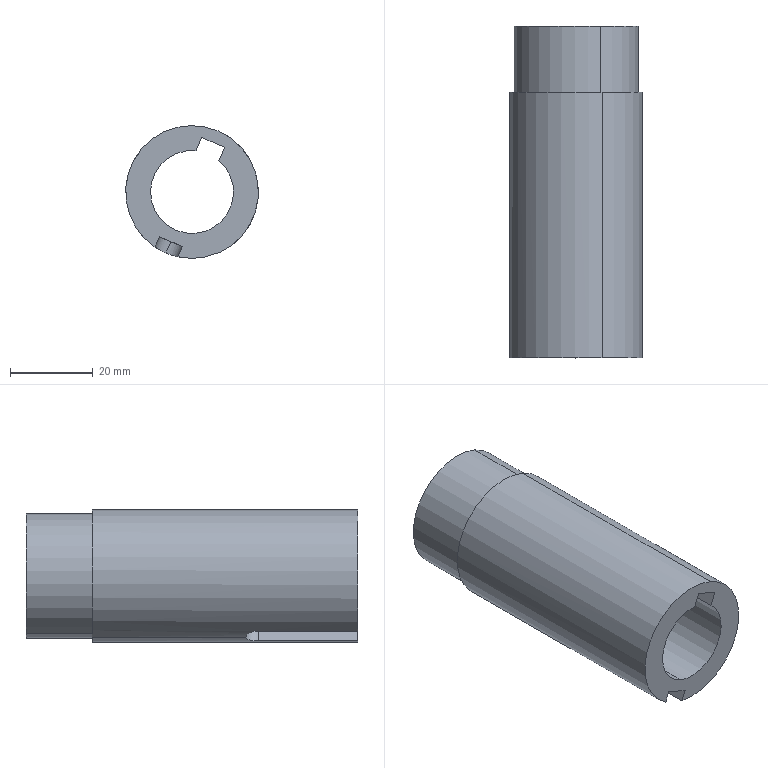Component | SolidWorks | -MovingSleeve-1 | 1 solid | 17 faces | box 32 x 80 x 32 mm | volume 35676 mm3 | plane 9 | cylinder 8 | commonest cylinder face diameters 6 x2 32 x2 30 x2 20 x2
build123d program:
from build123d import *

# Parameters (mm, degrees)
CUT_EXTRUDE1_DEPTH = 3
SKETCH3_W          = 6.215
SKETCH3_H          = 6
CUT_EXTRUDE2_DEPTH = 84.138


with BuildPart() as part:
    # Sketch1 → Revolve1 (revolve)
    with BuildSketch(Plane.XY):
        Polygon((15, 80), (15, 64), (16, 64), (16, 48), (16, 38), (16, 0), (10, 0), (10, 80), align=None)
    revolve(axis=Axis((0, -3319.583, 0), (0, 1, 0)))

    # Sketch2 → Cut-Extrude1 (cut)
    with BuildSketch(Plane(origin=(16, 0, 0), x_dir=(0, 0, -1), z_dir=(1, 0, 0))):
        with BuildLine():
            Line((-3, 0), (-3, 24))
            ThreePointArc((-3, 24), (0, 27), (3, 24))
            Line((3, 24), (3, 0))
            ThreePointArc((3, 0), (0, -3), (-3, 0))
        make_face()
    extrude(amount=-CUT_EXTRUDE1_DEPTH, mode=Mode.SUBTRACT)

    # Sketch3 → Cut-Extrude2 (cut, through all)
    with BuildSketch(Plane.XZ):
        with Locations((-9.893, 0)):
            Rectangle(SKETCH3_W, SKETCH3_H)
    extrude(amount=-CUT_EXTRUDE2_DEPTH, mode=Mode.SUBTRACT)


solid = part.part

# Placed as in the assembly
solid = solid.moved(Location((205, 1261.878, -173), (180, 66.949, -180)))
STEP:
#1=COLOUR_RGB('',0.7922,0.8196,0.9333);
#2=FILL_AREA_STYLE_COLOUR('',#1);
#3=FILL_AREA_STYLE('',(#2));
#4=SURFACE_STYLE_FILL_AREA(#3);
#5=SURFACE_SIDE_STYLE('',(#4));
#6=SURFACE_STYLE_USAGE(.BOTH.,#5);
#7=PRESENTATION_STYLE_ASSIGNMENT((#6));
#8=CARTESIAN_POINT('',(7.87,50.743,-7.282));
#9=VERTEX_POINT('',#8);
#10=CARTESIAN_POINT('',(7.979,50.625,-7.328));
#11=VERTEX_POINT('',#10);
#12=CARTESIAN_POINT('',(7.87,50.625,-7.282));
#13=DIRECTION('',(-0.3916,0.,-0.9202));
#14=DIRECTION('',(0.,1.,0.));
#15=AXIS2_PLACEMENT_3D('',#12,#13,#14);
#16=CIRCLE('',#15,0.1181);
#17=EDGE_CURVE('',#9,#11,#16,.T.);
#18=ORIENTED_EDGE('',*,*,#17,.F.);
#19=CARTESIAN_POINT('',(7.824,50.743,-7.391));
#20=VERTEX_POINT('',#19);
#21=CARTESIAN_POINT('',(7.87,50.743,-7.282));
#22=DIRECTION('',(-0.3916,0.,-0.9202));
#23=VECTOR('',#22,39.37);
#24=LINE('',#21,#23);
#25=EDGE_CURVE('',#9,#20,#24,.T.);
#26=ORIENTED_EDGE('',*,*,#25,.T.);
#27=CARTESIAN_POINT('',(7.937,50.625,-7.427));
#28=VERTEX_POINT('',#27);
#29=CARTESIAN_POINT('',(7.824,50.743,-7.391));
#30=CARTESIAN_POINT('',(7.831,50.743,-7.394));
#31=CARTESIAN_POINT('',(7.839,50.742,-7.397));
#32=CARTESIAN_POINT('',(7.853,50.739,-7.402));
#33=CARTESIAN_POINT('',(7.86,50.737,-7.405));
#34=CARTESIAN_POINT('',(7.873,50.731,-7.409));
#35=CARTESIAN_POINT('',(7.88,50.728,-7.411));
#36=CARTESIAN_POINT('',(7.892,50.719,-7.415));
#37=CARTESIAN_POINT('',(7.898,50.714,-7.417));
#38=CARTESIAN_POINT('',(7.909,50.703,-7.42));
#39=CARTESIAN_POINT('',(7.913,50.697,-7.421));
#40=CARTESIAN_POINT('',(7.922,50.684,-7.423));
#41=CARTESIAN_POINT('',(7.925,50.678,-7.424));
#42=CARTESIAN_POINT('',(7.931,50.663,-7.425));
#43=CARTESIAN_POINT('',(7.933,50.656,-7.426));
#44=CARTESIAN_POINT('',(7.936,50.641,-7.426));
#45=CARTESIAN_POINT('',(7.937,50.633,-7.427));
#46=CARTESIAN_POINT('',(7.937,50.625,-7.427));
#47=B_SPLINE_CURVE_WITH_KNOTS('',3,(#29,#30,#31,#32,#33,#34,#35,#36,#37,#38,#39,#40,#41,#42,#43,#44,#45,#46),.UNSPECIFIED.,.F.,.F.,(4,2,2,2,2,2,2,2,4),(0.004701,0.005288,0.005875,0.006462,0.007049,0.007637,0.008224,0.008811,0.009398),.UNSPECIFIED.);
#48=EDGE_CURVE('',#20,#28,#47,.T.);
#49=ORIENTED_EDGE('',*,*,#48,.T.);
#50=CARTESIAN_POINT('',(7.979,50.625,-7.328));
#51=DIRECTION('',(-0.3916,0.,-0.9202));
#52=VECTOR('',#51,39.37);
#53=LINE('',#50,#52);
#54=EDGE_CURVE('',#11,#28,#53,.T.);
#55=ORIENTED_EDGE('',*,*,#54,.F.);
#56=EDGE_LOOP('',(#18,#26,#49,#55));
#57=FACE_OUTER_BOUND('',#56,.T.);
#58=CARTESIAN_POINT('',(7.87,50.625,-7.282));
#59=DIRECTION('',(-0.3916,0.,-0.9202));
#60=DIRECTION('',(0.,1.,0.));
#61=AXIS2_PLACEMENT_3D('',#58,#59,#60);
#62=CYLINDRICAL_SURFACE('',#61,0.1181);
#63=ADVANCED_FACE('',(#57),#62,.F.);
#64=CARTESIAN_POINT('',(7.824,52.2,-7.391));
#65=VERTEX_POINT('',#64);
#66=CARTESIAN_POINT('',(8.318,52.2,-6.231));
#67=VERTEX_POINT('',#66);
#68=CARTESIAN_POINT('',(8.071,52.2,-6.811));
#69=DIRECTION('',(-0.,-1.,-0.));
#70=DIRECTION('',(-0.3916,0.,-0.9202));
#71=AXIS2_PLACEMENT_3D('',#68,#69,#70);
#72=CIRCLE('',#71,0.6299);
#73=EDGE_CURVE('',#65,#67,#72,.T.);
#74=ORIENTED_EDGE('',*,*,#73,.T.);
#75=CARTESIAN_POINT('',(8.318,49.68,-6.231));
#76=VERTEX_POINT('',#75);
#77=CARTESIAN_POINT('',(8.318,-81.012,-6.231));
#78=DIRECTION('',(-0.,-1.,-0.));
#79=VECTOR('',#78,39.37);
#80=LINE('',#77,#79);
#81=EDGE_CURVE('',#67,#76,#80,.T.);
#82=ORIENTED_EDGE('',*,*,#81,.T.);
#83=CARTESIAN_POINT('',(7.937,49.68,-7.427));
#84=VERTEX_POINT('',#83);
#85=CARTESIAN_POINT('',(8.071,49.68,-6.811));
#86=DIRECTION('',(-0.,-1.,-0.));
#87=DIRECTION('',(-0.3916,0.,-0.9202));
#88=AXIS2_PLACEMENT_3D('',#85,#86,#87);
#89=CIRCLE('',#88,0.6299);
#90=EDGE_CURVE('',#84,#76,#89,.T.);
#91=ORIENTED_EDGE('',*,*,#90,.F.);
#92=CARTESIAN_POINT('',(7.937,-81.012,-7.427));
#93=DIRECTION('',(-0.,-1.,-0.));
#94=VECTOR('',#93,39.37);
#95=LINE('',#92,#94);
#96=EDGE_CURVE('',#28,#84,#95,.T.);
#97=ORIENTED_EDGE('',*,*,#96,.F.);
#98=ORIENTED_EDGE('',*,*,#48,.F.);
#99=CARTESIAN_POINT('',(7.824,-81.012,-7.391));
#100=DIRECTION('',(-0.,-1.,-0.));
#101=VECTOR('',#100,39.37);
#102=LINE('',#99,#101);
#103=EDGE_CURVE('',#65,#20,#102,.T.);
#104=ORIENTED_EDGE('',*,*,#103,.F.);
#105=EDGE_LOOP('',(#74,#82,#91,#97,#98,#104));
#106=FACE_OUTER_BOUND('',#105,.T.);
#107=CARTESIAN_POINT('',(8.071,-81.012,-6.811));
#108=DIRECTION('',(-0.,-1.,-0.));
#109=DIRECTION('',(-0.3916,0.,-0.9202));
#110=AXIS2_PLACEMENT_3D('',#107,#108,#109);
#111=CYLINDRICAL_SURFACE('',#110,0.6299);
#112=ADVANCED_FACE('',(#106),#111,.T.);
#113=CARTESIAN_POINT('',(7.84,52.83,-7.354));
#114=VERTEX_POINT('',#113);
#115=CARTESIAN_POINT('',(8.302,52.83,-6.268));
#116=VERTEX_POINT('',#115);
#117=CARTESIAN_POINT('',(8.071,52.83,-6.811));
#118=DIRECTION('',(-0.,-1.,-0.));
#119=DIRECTION('',(-0.3916,0.,-0.9202));
#120=AXIS2_PLACEMENT_3D('',#117,#118,#119);
#121=CIRCLE('',#120,0.5906);
#122=EDGE_CURVE('',#114,#116,#121,.T.);
#123=ORIENTED_EDGE('',*,*,#122,.T.);
#124=CARTESIAN_POINT('',(8.302,52.2,-6.268));
#125=VERTEX_POINT('',#124);
#126=CARTESIAN_POINT('',(8.302,-81.012,-6.268));
#127=DIRECTION('',(-0.,-1.,-0.));
#128=VECTOR('',#127,39.37);
#129=LINE('',#126,#128);
#130=EDGE_CURVE('',#116,#125,#129,.T.);
#131=ORIENTED_EDGE('',*,*,#130,.T.);
#132=CARTESIAN_POINT('',(7.84,52.2,-7.354));
#133=VERTEX_POINT('',#132);
#134=CARTESIAN_POINT('',(8.071,52.2,-6.811));
#135=DIRECTION('',(-0.,-1.,-0.));
#136=DIRECTION('',(-0.3916,0.,-0.9202));
#137=AXIS2_PLACEMENT_3D('',#134,#135,#136);
#138=CIRCLE('',#137,0.5906);
#139=EDGE_CURVE('',#133,#125,#138,.T.);
#140=ORIENTED_EDGE('',*,*,#139,.F.);
#141=CARTESIAN_POINT('',(7.84,-81.012,-7.354));
#142=DIRECTION('',(-0.,-1.,-0.));
#143=VECTOR('',#142,39.37);
#144=LINE('',#141,#143);
#145=EDGE_CURVE('',#114,#133,#144,.T.);
#146=ORIENTED_EDGE('',*,*,#145,.F.);
#147=EDGE_LOOP('',(#123,#131,#140,#146));
#148=FACE_OUTER_BOUND('',#147,.T.);
#149=CARTESIAN_POINT('',(8.071,-81.012,-6.811));
#150=DIRECTION('',(-0.,-1.,-0.));
#151=DIRECTION('',(-0.3916,0.,-0.9202));
#152=AXIS2_PLACEMENT_3D('',#149,#150,#151);
#153=CYLINDRICAL_SURFACE('',#152,0.5906);
#154=ADVANCED_FACE('',(#148),#153,.T.);
#155=CARTESIAN_POINT('',(7.917,52.83,-7.173));
#156=VERTEX_POINT('',#155);
#157=CARTESIAN_POINT('',(8.327,52.83,-6.512));
#158=VERTEX_POINT('',#157);
#159=CARTESIAN_POINT('',(8.071,52.83,-6.811));
#160=DIRECTION('',(-0.,-1.,-0.));
#161=DIRECTION('',(-0.3916,0.,-0.9202));
#162=AXIS2_PLACEMENT_3D('',#159,#160,#161);
#163=CIRCLE('',#162,0.3937);
#164=EDGE_CURVE('',#156,#158,#163,.T.);
#165=ORIENTED_EDGE('',*,*,#164,.F.);
#166=CARTESIAN_POINT('',(7.917,49.68,-7.173));
#167=VERTEX_POINT('',#166);
#168=CARTESIAN_POINT('',(7.917,-81.012,-7.173));
#169=DIRECTION('',(-0.,-1.,-0.));
#170=VECTOR('',#169,39.37);
#171=LINE('',#168,#170);
#172=EDGE_CURVE('',#156,#167,#171,.T.);
#173=ORIENTED_EDGE('',*,*,#172,.T.);
#174=CARTESIAN_POINT('',(8.327,49.68,-6.512));
#175=VERTEX_POINT('',#174);
#176=CARTESIAN_POINT('',(8.071,49.68,-6.811));
#177=DIRECTION('',(-0.,-1.,-0.));
#178=DIRECTION('',(-0.3916,0.,-0.9202));
#179=AXIS2_PLACEMENT_3D('',#176,#177,#178);
#180=CIRCLE('',#179,0.3937);
#181=EDGE_CURVE('',#167,#175,#180,.T.);
#182=ORIENTED_EDGE('',*,*,#181,.T.);
#183=CARTESIAN_POINT('',(8.327,-81.012,-6.512));
#184=DIRECTION('',(-0.,-1.,-0.));
#185=VECTOR('',#184,39.37);
#186=LINE('',#183,#185);
#187=EDGE_CURVE('',#158,#175,#186,.T.);
#188=ORIENTED_EDGE('',*,*,#187,.F.);
#189=EDGE_LOOP('',(#165,#173,#182,#188));
#190=FACE_OUTER_BOUND('',#189,.T.);
#191=CARTESIAN_POINT('',(8.071,-81.012,-6.811));
#192=DIRECTION('',(-0.,-1.,-0.));
#193=DIRECTION('',(-0.3916,0.,-0.9202));
#194=AXIS2_PLACEMENT_3D('',#191,#192,#193);
#195=CYLINDRICAL_SURFACE('',#194,0.3937);
#196=ADVANCED_FACE('',(#190),#195,.F.);
#197=ORIENTED_EDGE('',*,*,#172,.F.);
#198=CARTESIAN_POINT('',(8.109,52.83,-6.419));
#199=VERTEX_POINT('',#198);
#200=CARTESIAN_POINT('',(8.071,52.83,-6.811));
#201=DIRECTION('',(-0.,-1.,-0.));
#202=DIRECTION('',(-0.3916,0.,-0.9202));
#203=AXIS2_PLACEMENT_3D('',#200,#201,#202);
#204=CIRCLE('',#203,0.3937);
#205=EDGE_CURVE('',#199,#156,#204,.T.);
#206=ORIENTED_EDGE('',*,*,#205,.F.);
#207=CARTESIAN_POINT('',(8.109,49.68,-6.419));
#208=VERTEX_POINT('',#207);
#209=CARTESIAN_POINT('',(8.109,-81.012,-6.419));
#210=DIRECTION('',(0.,1.,0.));
#211=VECTOR('',#210,39.37);
#212=LINE('',#209,#211);
#213=EDGE_CURVE('',#208,#199,#212,.T.);
#214=ORIENTED_EDGE('',*,*,#213,.F.);
#215=CARTESIAN_POINT('',(8.071,49.68,-6.811));
#216=DIRECTION('',(-0.,-1.,-0.));
#217=DIRECTION('',(-0.3916,0.,-0.9202));
#218=AXIS2_PLACEMENT_3D('',#215,#216,#217);
#219=CIRCLE('',#218,0.3937);
#220=EDGE_CURVE('',#208,#167,#219,.T.);
#221=ORIENTED_EDGE('',*,*,#220,.T.);
#222=EDGE_LOOP('',(#197,#206,#214,#221));
#223=FACE_OUTER_BOUND('',#222,.T.);
#224=CARTESIAN_POINT('',(8.071,-81.012,-6.811));
#225=DIRECTION('',(-0.,-1.,-0.));
#226=DIRECTION('',(-0.3916,0.,-0.9202));
#227=AXIS2_PLACEMENT_3D('',#224,#225,#226);
#228=CYLINDRICAL_SURFACE('',#227,0.3937);
#229=ADVANCED_FACE('',(#223),#228,.F.);
#230=CARTESIAN_POINT('',(8.38,52.83,-6.386));
#231=VERTEX_POINT('',#230);
#232=CARTESIAN_POINT('',(8.38,52.83,-6.386));
#233=DIRECTION('',(0.3916,-0.,0.9202));
#234=VECTOR('',#233,39.37);
#235=LINE('',#232,#234);
#236=EDGE_CURVE('',#158,#231,#235,.T.);
#237=ORIENTED_EDGE('',*,*,#236,.T.);
#238=CARTESIAN_POINT('',(8.163,52.83,-6.294));
#239=VERTEX_POINT('',#238);
#240=CARTESIAN_POINT('',(8.38,52.83,-6.386));
#241=DIRECTION('',(-0.9202,0.,0.3916));
#242=VECTOR('',#241,39.37);
#243=LINE('',#240,#242);
#244=EDGE_CURVE('',#231,#239,#243,.T.);
#245=ORIENTED_EDGE('',*,*,#244,.T.);
#246=CARTESIAN_POINT('',(8.163,52.83,-6.294));
#247=DIRECTION('',(-0.3916,0.,-0.9202));
#248=VECTOR('',#247,39.37);
#249=LINE('',#246,#248);
#250=EDGE_CURVE('',#239,#199,#249,.T.);
#251=ORIENTED_EDGE('',*,*,#250,.T.);
#252=ORIENTED_EDGE('',*,*,#205,.T.);
#253=ORIENTED_EDGE('',*,*,#164,.T.);
#254=EDGE_LOOP('',(#237,#245,#251,#252,#253));
#255=FACE_BOUND('',#254,.T.);
#256=ORIENTED_EDGE('',*,*,#122,.F.);
#257=CARTESIAN_POINT('',(8.071,52.83,-6.811));
#258=DIRECTION('',(-0.,-1.,-0.));
#259=DIRECTION('',(-0.3916,0.,-0.9202));
#260=AXIS2_PLACEMENT_3D('',#257,#258,#259);
#261=CIRCLE('',#260,0.5906);
#262=EDGE_CURVE('',#116,#114,#261,.T.);
#263=ORIENTED_EDGE('',*,*,#262,.F.);
#264=EDGE_LOOP('',(#256,#263));
#265=FACE_OUTER_BOUND('',#264,.T.);
#266=CARTESIAN_POINT('',(7.917,52.83,-7.173));
#267=DIRECTION('',(0.,1.,0.));
#268=DIRECTION('',(0.3916,-0.,0.9202));
#269=AXIS2_PLACEMENT_3D('',#266,#267,#268);
#270=PLANE('',#269);
#271=ADVANCED_FACE('',(#255,#265),#270,.T.);
#272=ORIENTED_EDGE('',*,*,#130,.F.);
#273=ORIENTED_EDGE('',*,*,#262,.T.);
#274=ORIENTED_EDGE('',*,*,#145,.T.);
#275=CARTESIAN_POINT('',(8.071,52.2,-6.811));
#276=DIRECTION('',(-0.,-1.,-0.));
#277=DIRECTION('',(-0.3916,0.,-0.9202));
#278=AXIS2_PLACEMENT_3D('',#275,#276,#277);
#279=CIRCLE('',#278,0.5906);
#280=EDGE_CURVE('',#125,#133,#279,.T.);
#281=ORIENTED_EDGE('',*,*,#280,.F.);
#282=EDGE_LOOP('',(#272,#273,#274,#281));
#283=FACE_OUTER_BOUND('',#282,.T.);
#284=CARTESIAN_POINT('',(8.071,-81.012,-6.811));
#285=DIRECTION('',(-0.,-1.,-0.));
#286=DIRECTION('',(-0.3916,0.,-0.9202));
#287=AXIS2_PLACEMENT_3D('',#284,#285,#286);
#288=CYLINDRICAL_SURFACE('',#287,0.5906);
#289=ADVANCED_FACE('',(#283),#288,.T.);
#290=ORIENTED_EDGE('',*,*,#139,.T.);
#291=ORIENTED_EDGE('',*,*,#280,.T.);
#292=EDGE_LOOP('',(#290,#291));
#293=FACE_BOUND('',#292,.T.);
#294=ORIENTED_EDGE('',*,*,#73,.F.);
#295=CARTESIAN_POINT('',(8.071,52.2,-6.811));
#296=DIRECTION('',(-0.,-1.,-0.));
#297=DIRECTION('',(-0.3916,0.,-0.9202));
#298=AXIS2_PLACEMENT_3D('',#295,#296,#297);
#299=CIRCLE('',#298,0.6299);
#300=EDGE_CURVE('',#67,#65,#299,.T.);
#301=ORIENTED_EDGE('',*,*,#300,.F.);
#302=EDGE_LOOP('',(#294,#301));
#303=FACE_OUTER_BOUND('',#302,.T.);
#304=CARTESIAN_POINT('',(7.84,52.2,-7.354));
#305=DIRECTION('',(0.,1.,0.));
#306=DIRECTION('',(0.3916,-0.,0.9202));
#307=AXIS2_PLACEMENT_3D('',#304,#305,#306);
#308=PLANE('',#307);
#309=ADVANCED_FACE('',(#293,#303),#308,.T.);
#310=ORIENTED_EDGE('',*,*,#81,.F.);
#311=ORIENTED_EDGE('',*,*,#300,.T.);
#312=ORIENTED_EDGE('',*,*,#103,.T.);
#313=CARTESIAN_POINT('',(7.72,50.625,-7.334));
#314=VERTEX_POINT('',#313);
#315=CARTESIAN_POINT('',(7.72,50.625,-7.334));
#316=CARTESIAN_POINT('',(7.72,50.633,-7.334));
#317=CARTESIAN_POINT('',(7.721,50.641,-7.335));
#318=CARTESIAN_POINT('',(7.723,50.656,-7.336));
#319=CARTESIAN_POINT('',(7.725,50.663,-7.338));
#320=CARTESIAN_POINT('',(7.73,50.678,-7.341));
#321=CARTESIAN_POINT('',(7.733,50.684,-7.343));
#322=CARTESIAN_POINT('',(7.741,50.697,-7.347));
#323=CARTESIAN_POINT('',(7.745,50.703,-7.35));
#324=CARTESIAN_POINT('',(7.754,50.714,-7.356));
#325=CARTESIAN_POINT('',(7.759,50.719,-7.359));
#326=CARTESIAN_POINT('',(7.771,50.728,-7.365));
#327=CARTESIAN_POINT('',(7.777,50.731,-7.368));
#328=CARTESIAN_POINT('',(7.79,50.737,-7.375));
#329=CARTESIAN_POINT('',(7.796,50.739,-7.378));
#330=CARTESIAN_POINT('',(7.81,50.742,-7.384));
#331=CARTESIAN_POINT('',(7.817,50.743,-7.388));
#332=CARTESIAN_POINT('',(7.824,50.743,-7.391));
#333=B_SPLINE_CURVE_WITH_KNOTS('',3,(#315,#316,#317,#318,#319,#320,#321,#322,#323,#324,#325,#326,#327,#328,#329,#330,#331,#332),.UNSPECIFIED.,.F.,.F.,(4,2,2,2,2,2,2,2,4),(0.,0.0005877,0.001175,0.001763,0.002351,0.002938,0.003526,0.004114,0.004701),.UNSPECIFIED.);
#334=EDGE_CURVE('',#314,#20,#333,.T.);
#335=ORIENTED_EDGE('',*,*,#334,.F.);
#336=CARTESIAN_POINT('',(7.72,49.68,-7.334));
#337=VERTEX_POINT('',#336);
#338=CARTESIAN_POINT('',(7.72,-81.012,-7.334));
#339=DIRECTION('',(0.,1.,0.));
#340=VECTOR('',#339,39.37);
#341=LINE('',#338,#340);
#342=EDGE_CURVE('',#337,#314,#341,.T.);
#343=ORIENTED_EDGE('',*,*,#342,.F.);
#344=CARTESIAN_POINT('',(8.071,49.68,-6.811));
#345=DIRECTION('',(-0.,-1.,-0.));
#346=DIRECTION('',(-0.3916,0.,-0.9202));
#347=AXIS2_PLACEMENT_3D('',#344,#345,#346);
#348=CIRCLE('',#347,0.6299);
#349=EDGE_CURVE('',#76,#337,#348,.T.);
#350=ORIENTED_EDGE('',*,*,#349,.F.);
#351=EDGE_LOOP('',(#310,#311,#312,#335,#343,#350));
#352=FACE_OUTER_BOUND('',#351,.T.);
#353=CARTESIAN_POINT('',(8.071,-81.012,-6.811));
#354=DIRECTION('',(-0.,-1.,-0.));
#355=DIRECTION('',(-0.3916,0.,-0.9202));
#356=AXIS2_PLACEMENT_3D('',#353,#354,#355);
#357=CYLINDRICAL_SURFACE('',#356,0.6299);
#358=ADVANCED_FACE('',(#352),#357,.T.);
#359=CARTESIAN_POINT('',(8.38,49.68,-6.386));
#360=VERTEX_POINT('',#359);
#361=CARTESIAN_POINT('',(8.025,49.68,-7.22));
#362=DIRECTION('',(0.3916,-0.,0.9202));
#363=VECTOR('',#362,39.37);
#364=LINE('',#361,#363);
#365=EDGE_CURVE('',#175,#360,#364,.T.);
#366=ORIENTED_EDGE('',*,*,#365,.F.);
#367=ORIENTED_EDGE('',*,*,#181,.F.);
#368=ORIENTED_EDGE('',*,*,#220,.F.);
#369=CARTESIAN_POINT('',(8.163,49.68,-6.294));
#370=VERTEX_POINT('',#369);
#371=CARTESIAN_POINT('',(8.163,49.68,-6.294));
#372=DIRECTION('',(-0.3916,0.,-0.9202));
#373=VECTOR('',#372,39.37);
#374=LINE('',#371,#373);
#375=EDGE_CURVE('',#370,#208,#374,.T.);
#376=ORIENTED_EDGE('',*,*,#375,.F.);
#377=CARTESIAN_POINT('',(8.38,49.68,-6.386));
#378=DIRECTION('',(-0.9202,0.,0.3916));
#379=VECTOR('',#378,39.37);
#380=LINE('',#377,#379);
#381=EDGE_CURVE('',#360,#370,#380,.T.);
#382=ORIENTED_EDGE('',*,*,#381,.F.);
#383=EDGE_LOOP('',(#366,#367,#368,#376,#382));
#384=FACE_BOUND('',#383,.T.);
#385=CARTESIAN_POINT('',(7.979,49.68,-7.328));
#386=VERTEX_POINT('',#385);
#387=CARTESIAN_POINT('',(7.979,49.68,-7.328));
#388=DIRECTION('',(-0.3916,0.,-0.9202));
#389=VECTOR('',#388,39.37);
#390=LINE('',#387,#389);
#391=EDGE_CURVE('',#386,#84,#390,.T.);
#392=ORIENTED_EDGE('',*,*,#391,.T.);
#393=ORIENTED_EDGE('',*,*,#90,.T.);
#394=ORIENTED_EDGE('',*,*,#349,.T.);
#395=CARTESIAN_POINT('',(7.762,49.68,-7.236));
#396=VERTEX_POINT('',#395);
#397=CARTESIAN_POINT('',(7.762,49.68,-7.236));
#398=DIRECTION('',(-0.3916,0.,-0.9202));
#399=VECTOR('',#398,39.37);
#400=LINE('',#397,#399);
#401=EDGE_CURVE('',#396,#337,#400,.T.);
#402=ORIENTED_EDGE('',*,*,#401,.F.);
#403=CARTESIAN_POINT('',(7.87,49.68,-7.282));
#404=DIRECTION('',(0.9202,-0.,-0.3916));
#405=VECTOR('',#404,39.37);
#406=LINE('',#403,#405);
#407=EDGE_CURVE('',#396,#386,#406,.T.);
#408=ORIENTED_EDGE('',*,*,#407,.T.);
#409=EDGE_LOOP('',(#392,#393,#394,#402,#408));
#410=FACE_OUTER_BOUND('',#409,.T.);
#411=CARTESIAN_POINT('',(7.917,49.68,-7.173));
#412=DIRECTION('',(-0.,-1.,-0.));
#413=DIRECTION('',(-0.3916,0.,-0.9202));
#414=AXIS2_PLACEMENT_3D('',#411,#412,#413);
#415=PLANE('',#414);
#416=ADVANCED_FACE('',(#384,#410),#415,.T.);
#417=ORIENTED_EDGE('',*,*,#96,.T.);
#418=ORIENTED_EDGE('',*,*,#391,.F.);
#419=CARTESIAN_POINT('',(7.979,49.68,-7.328));
#420=DIRECTION('',(0.,-1.,0.));
#421=VECTOR('',#420,39.37);
#422=LINE('',#419,#421);
#423=EDGE_CURVE('',#11,#386,#422,.T.);
#424=ORIENTED_EDGE('',*,*,#423,.F.);
#425=ORIENTED_EDGE('',*,*,#54,.T.);
#426=EDGE_LOOP('',(#417,#418,#424,#425));
#427=FACE_OUTER_BOUND('',#426,.T.);
#428=CARTESIAN_POINT('',(7.979,49.68,-7.328));
#429=DIRECTION('',(0.9202,-0.,-0.3916));
#430=DIRECTION('',(-0.3916,-0.,-0.9202));
#431=AXIS2_PLACEMENT_3D('',#428,#429,#430);
#432=PLANE('',#431);
#433=ADVANCED_FACE('',(#427),#432,.F.);
#434=ORIENTED_EDGE('',*,*,#25,.F.);
#435=CARTESIAN_POINT('',(7.762,50.625,-7.236));
#436=VERTEX_POINT('',#435);
#437=CARTESIAN_POINT('',(7.87,50.625,-7.282));
#438=DIRECTION('',(-0.3916,0.,-0.9202));
#439=DIRECTION('',(0.,1.,0.));
#440=AXIS2_PLACEMENT_3D('',#437,#438,#439);
#441=CIRCLE('',#440,0.1181);
#442=EDGE_CURVE('',#436,#9,#441,.T.);
#443=ORIENTED_EDGE('',*,*,#442,.F.);
#444=CARTESIAN_POINT('',(7.762,50.625,-7.236));
#445=DIRECTION('',(-0.3916,0.,-0.9202));
#446=VECTOR('',#445,39.37);
#447=LINE('',#444,#446);
#448=EDGE_CURVE('',#436,#314,#447,.T.);
#449=ORIENTED_EDGE('',*,*,#448,.T.);
#450=ORIENTED_EDGE('',*,*,#334,.T.);
#451=EDGE_LOOP('',(#434,#443,#449,#450));
#452=FACE_OUTER_BOUND('',#451,.T.);
#453=CARTESIAN_POINT('',(7.87,50.625,-7.282));
#454=DIRECTION('',(-0.3916,0.,-0.9202));
#455=DIRECTION('',(0.,1.,0.));
#456=AXIS2_PLACEMENT_3D('',#453,#454,#455);
#457=CYLINDRICAL_SURFACE('',#456,0.1181);
#458=ADVANCED_FACE('',(#452),#457,.F.);
#459=ORIENTED_EDGE('',*,*,#342,.T.);
#460=ORIENTED_EDGE('',*,*,#448,.F.);
#461=CARTESIAN_POINT('',(7.762,49.68,-7.236));
#462=DIRECTION('',(-0.,1.,-0.));
#463=VECTOR('',#462,39.37);
#464=LINE('',#461,#463);
#465=EDGE_CURVE('',#396,#436,#464,.T.);
#466=ORIENTED_EDGE('',*,*,#465,.F.);
#467=ORIENTED_EDGE('',*,*,#401,.T.);
#468=EDGE_LOOP('',(#459,#460,#466,#467));
#469=FACE_OUTER_BOUND('',#468,.T.);
#470=CARTESIAN_POINT('',(7.762,49.68,-7.236));
#471=DIRECTION('',(-0.9202,0.,0.3916));
#472=DIRECTION('',(0.3916,0.,0.9202));
#473=AXIS2_PLACEMENT_3D('',#470,#471,#472);
#474=PLANE('',#473);
#475=ADVANCED_FACE('',(#469),#474,.F.);
#476=ORIENTED_EDGE('',*,*,#465,.T.);
#477=ORIENTED_EDGE('',*,*,#442,.T.);
#478=ORIENTED_EDGE('',*,*,#17,.T.);
#479=ORIENTED_EDGE('',*,*,#423,.T.);
#480=ORIENTED_EDGE('',*,*,#407,.F.);
#481=EDGE_LOOP('',(#476,#477,#478,#479,#480));
#482=FACE_OUTER_BOUND('',#481,.T.);
#483=CARTESIAN_POINT('',(7.87,49.68,-7.282));
#484=DIRECTION('',(-0.3916,0.,-0.9202));
#485=DIRECTION('',(0.,1.,0.));
#486=AXIS2_PLACEMENT_3D('',#483,#484,#485);
#487=PLANE('',#486);
#488=ADVANCED_FACE('',(#482),#487,.T.);
#489=ORIENTED_EDGE('',*,*,#381,.T.);
#490=CARTESIAN_POINT('',(8.163,52.83,-6.294));
#491=DIRECTION('',(-0.,-1.,-0.));
#492=VECTOR('',#491,39.37);
#493=LINE('',#490,#492);
#494=EDGE_CURVE('',#239,#370,#493,.T.);
#495=ORIENTED_EDGE('',*,*,#494,.F.);
#496=ORIENTED_EDGE('',*,*,#244,.F.);
#497=CARTESIAN_POINT('',(8.38,52.83,-6.386));
#498=DIRECTION('',(-0.,-1.,-0.));
#499=VECTOR('',#498,39.37);
#500=LINE('',#497,#499);
#501=EDGE_CURVE('',#231,#360,#500,.T.);
#502=ORIENTED_EDGE('',*,*,#501,.T.);
#503=EDGE_LOOP('',(#489,#495,#496,#502));
#504=FACE_OUTER_BOUND('',#503,.T.);
#505=CARTESIAN_POINT('',(8.38,52.83,-6.386));
#506=DIRECTION('',(0.3916,-0.,0.9202));
#507=DIRECTION('',(-0.,-1.,-0.));
#508=AXIS2_PLACEMENT_3D('',#505,#506,#507);
#509=PLANE('',#508);
#510=ADVANCED_FACE('',(#504),#509,.F.);
#511=ORIENTED_EDGE('',*,*,#187,.T.);
#512=ORIENTED_EDGE('',*,*,#365,.T.);
#513=ORIENTED_EDGE('',*,*,#501,.F.);
#514=ORIENTED_EDGE('',*,*,#236,.F.);
#515=EDGE_LOOP('',(#511,#512,#513,#514));
#516=FACE_OUTER_BOUND('',#515,.T.);
#517=CARTESIAN_POINT('',(8.38,52.83,-6.386));
#518=DIRECTION('',(0.9202,-0.,-0.3916));
#519=DIRECTION('',(-0.3916,-0.,-0.9202));
#520=AXIS2_PLACEMENT_3D('',#517,#518,#519);
#521=PLANE('',#520);
#522=ADVANCED_FACE('',(#516),#521,.F.);
#523=ORIENTED_EDGE('',*,*,#213,.T.);
#524=ORIENTED_EDGE('',*,*,#250,.F.);
#525=ORIENTED_EDGE('',*,*,#494,.T.);
#526=ORIENTED_EDGE('',*,*,#375,.T.);
#527=EDGE_LOOP('',(#523,#524,#525,#526));
#528=FACE_OUTER_BOUND('',#527,.T.);
#529=CARTESIAN_POINT('',(8.163,52.83,-6.294));
#530=DIRECTION('',(-0.9202,0.,0.3916));
#531=DIRECTION('',(0.3916,0.,0.9202));
#532=AXIS2_PLACEMENT_3D('',#529,#530,#531);
#533=PLANE('',#532);
#534=ADVANCED_FACE('',(#528),#533,.F.);
#535=CLOSED_SHELL('',(#63,#112,#154,#196,#229,#271,#289,#309,#358,#416,#433,#458,#475,#488,#510,#522,#534));
#536=MANIFOLD_SOLID_BREP('',#535);
#537=STYLED_ITEM('',(#7),#536);
#538=(LENGTH_UNIT()NAMED_UNIT(*)SI_UNIT($,.METRE.));
#539=LENGTH_MEASURE_WITH_UNIT(LENGTH_MEASURE(0.0254),#538);
#540=DIMENSIONAL_EXPONENTS(1.,0.,0.,0.,0.,0.,0.);
#541=(CONVERSION_BASED_UNIT('',#539)LENGTH_UNIT()NAMED_UNIT(#540));
#542=UNCERTAINTY_MEASURE_WITH_UNIT(LENGTH_MEASURE(0.00001),#541,'','');
#543=(NAMED_UNIT(*)PLANE_ANGLE_UNIT()SI_UNIT($,.RADIAN.));
#544=(NAMED_UNIT(*)SI_UNIT($,.STERADIAN.)SOLID_ANGLE_UNIT());
#545=(GEOMETRIC_REPRESENTATION_CONTEXT(3)GLOBAL_UNCERTAINTY_ASSIGNED_CONTEXT((#542))GLOBAL_UNIT_ASSIGNED_CONTEXT((#541,#543,#544))REPRESENTATION_CONTEXT('',''));
#546=MECHANICAL_DESIGN_GEOMETRIC_PRESENTATION_REPRESENTATION('',(#537),#545);
#547=PRESENTATION_LAYER_ASSIGNMENT('','',(#537));
#548=CARTESIAN_POINT('',(0.,0.,0.));
#549=DIRECTION('',(0.,0.,1.));
#550=DIRECTION('',(1.,0.,0.));
#551=AXIS2_PLACEMENT_3D('',#548,#549,#550);
#552=(LENGTH_UNIT()NAMED_UNIT(*)SI_UNIT($,.METRE.));
#553=LENGTH_MEASURE_WITH_UNIT(LENGTH_MEASURE(0.0254),#552);
#554=DIMENSIONAL_EXPONENTS(1.,0.,0.,0.,0.,0.,0.);
#555=(CONVERSION_BASED_UNIT('',#553)LENGTH_UNIT()NAMED_UNIT(#554));
#556=UNCERTAINTY_MEASURE_WITH_UNIT(LENGTH_MEASURE(0.00001),#555,'','');
#557=(NAMED_UNIT(*)PLANE_ANGLE_UNIT()SI_UNIT($,.RADIAN.));
#558=(NAMED_UNIT(*)SI_UNIT($,.STERADIAN.)SOLID_ANGLE_UNIT());
#559=(GEOMETRIC_REPRESENTATION_CONTEXT(3)GLOBAL_UNCERTAINTY_ASSIGNED_CONTEXT((#556))GLOBAL_UNIT_ASSIGNED_CONTEXT((#555,#557,#558))REPRESENTATION_CONTEXT('',''));
#560=ADVANCED_BREP_SHAPE_REPRESENTATION('',(#536,#551),#559);